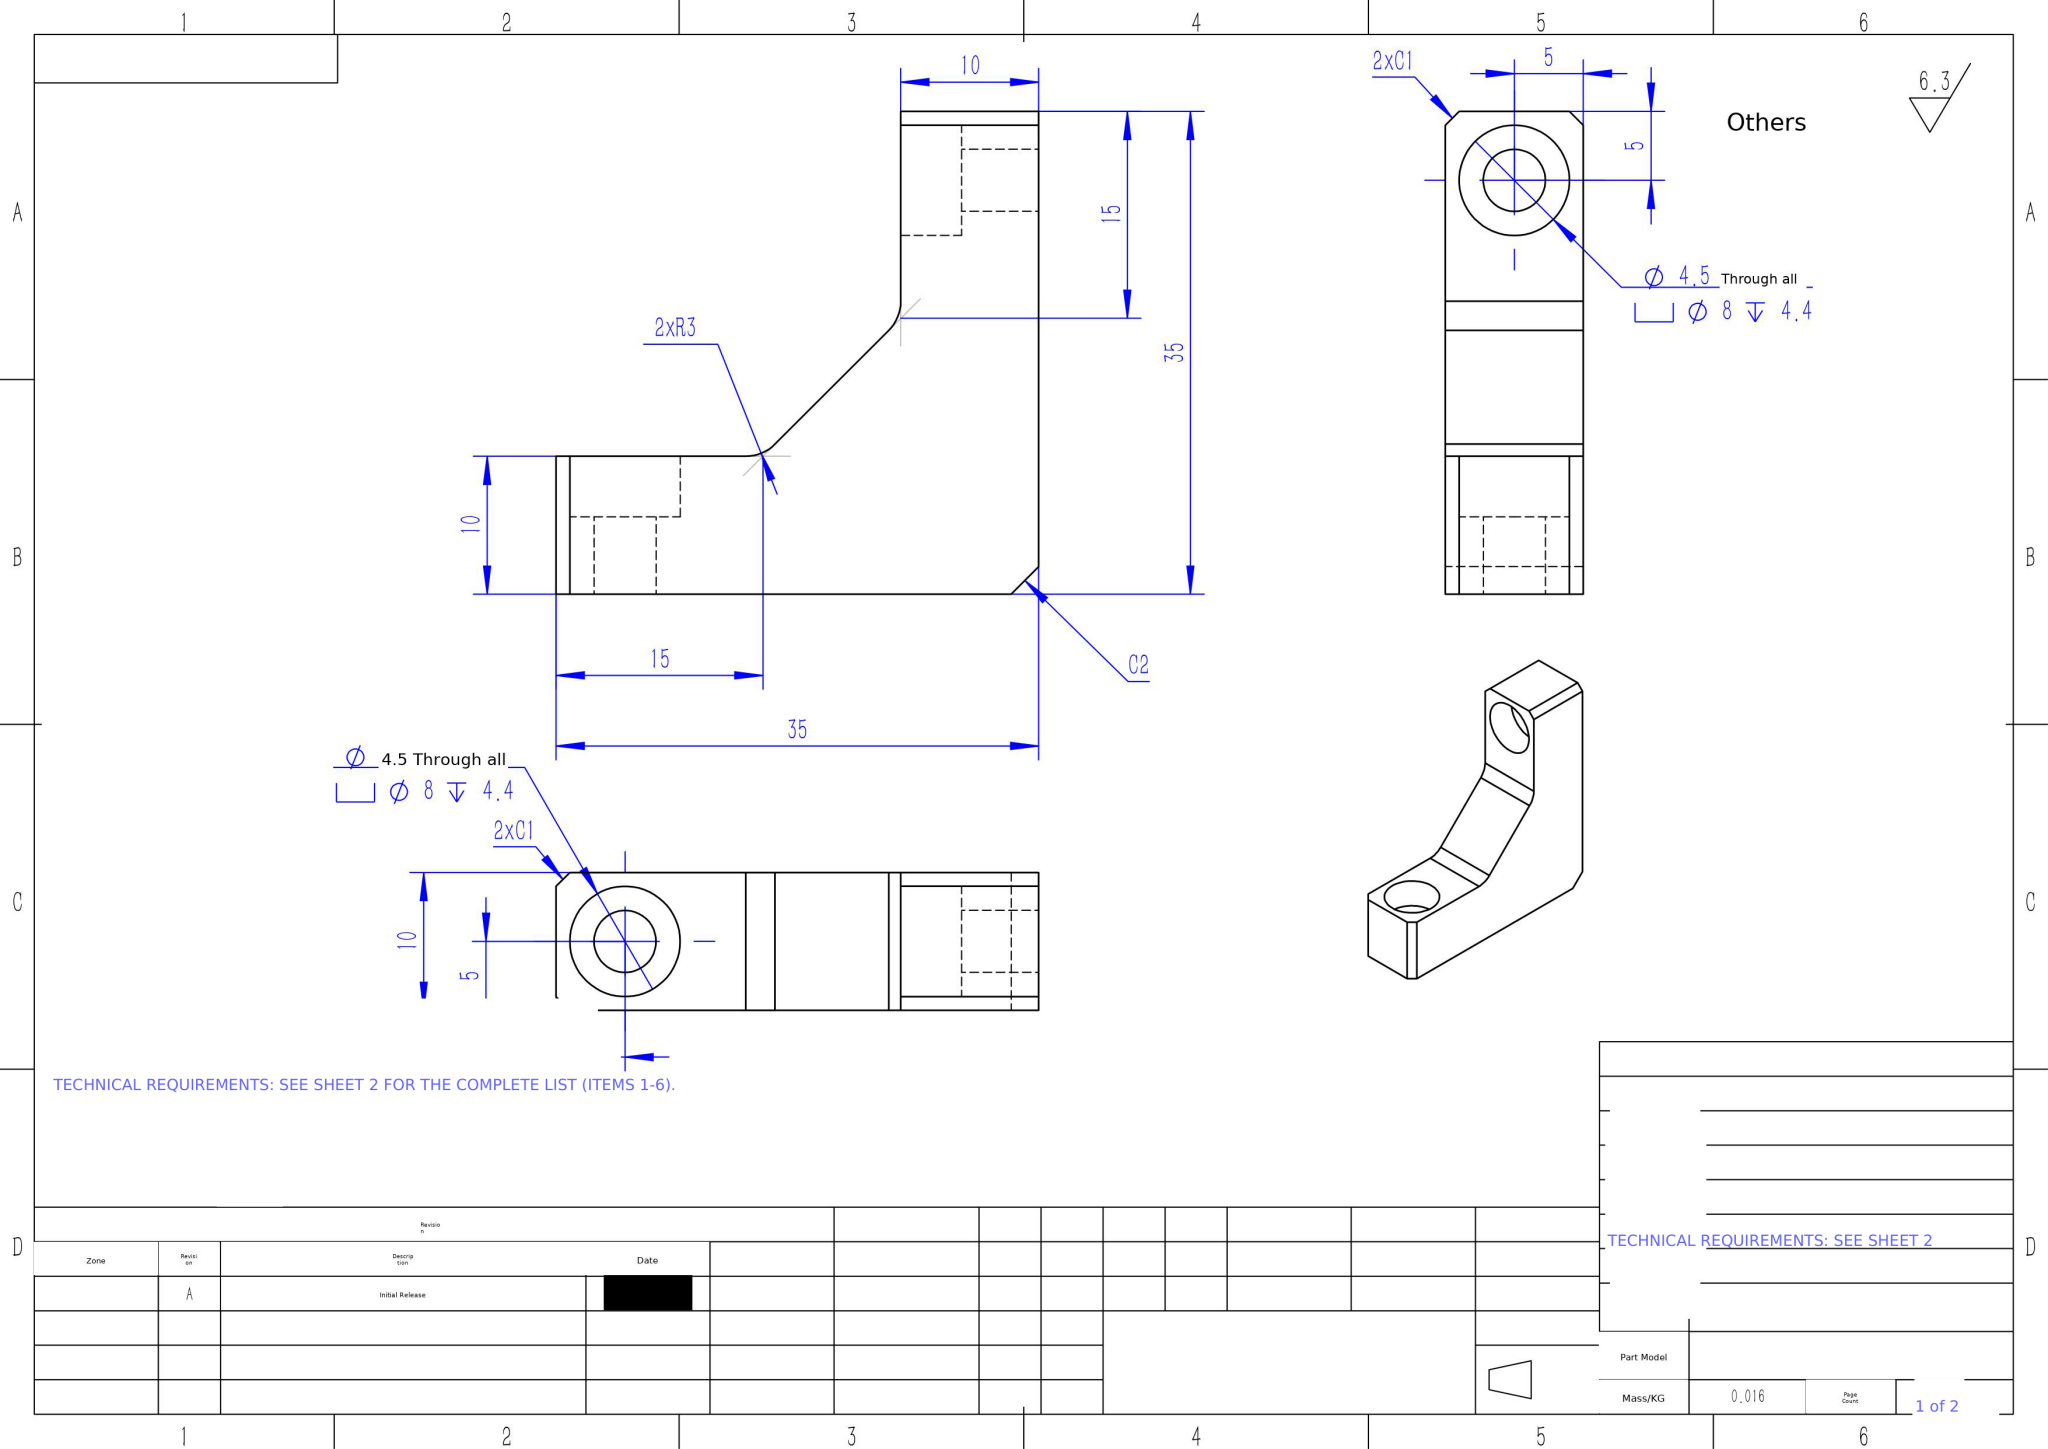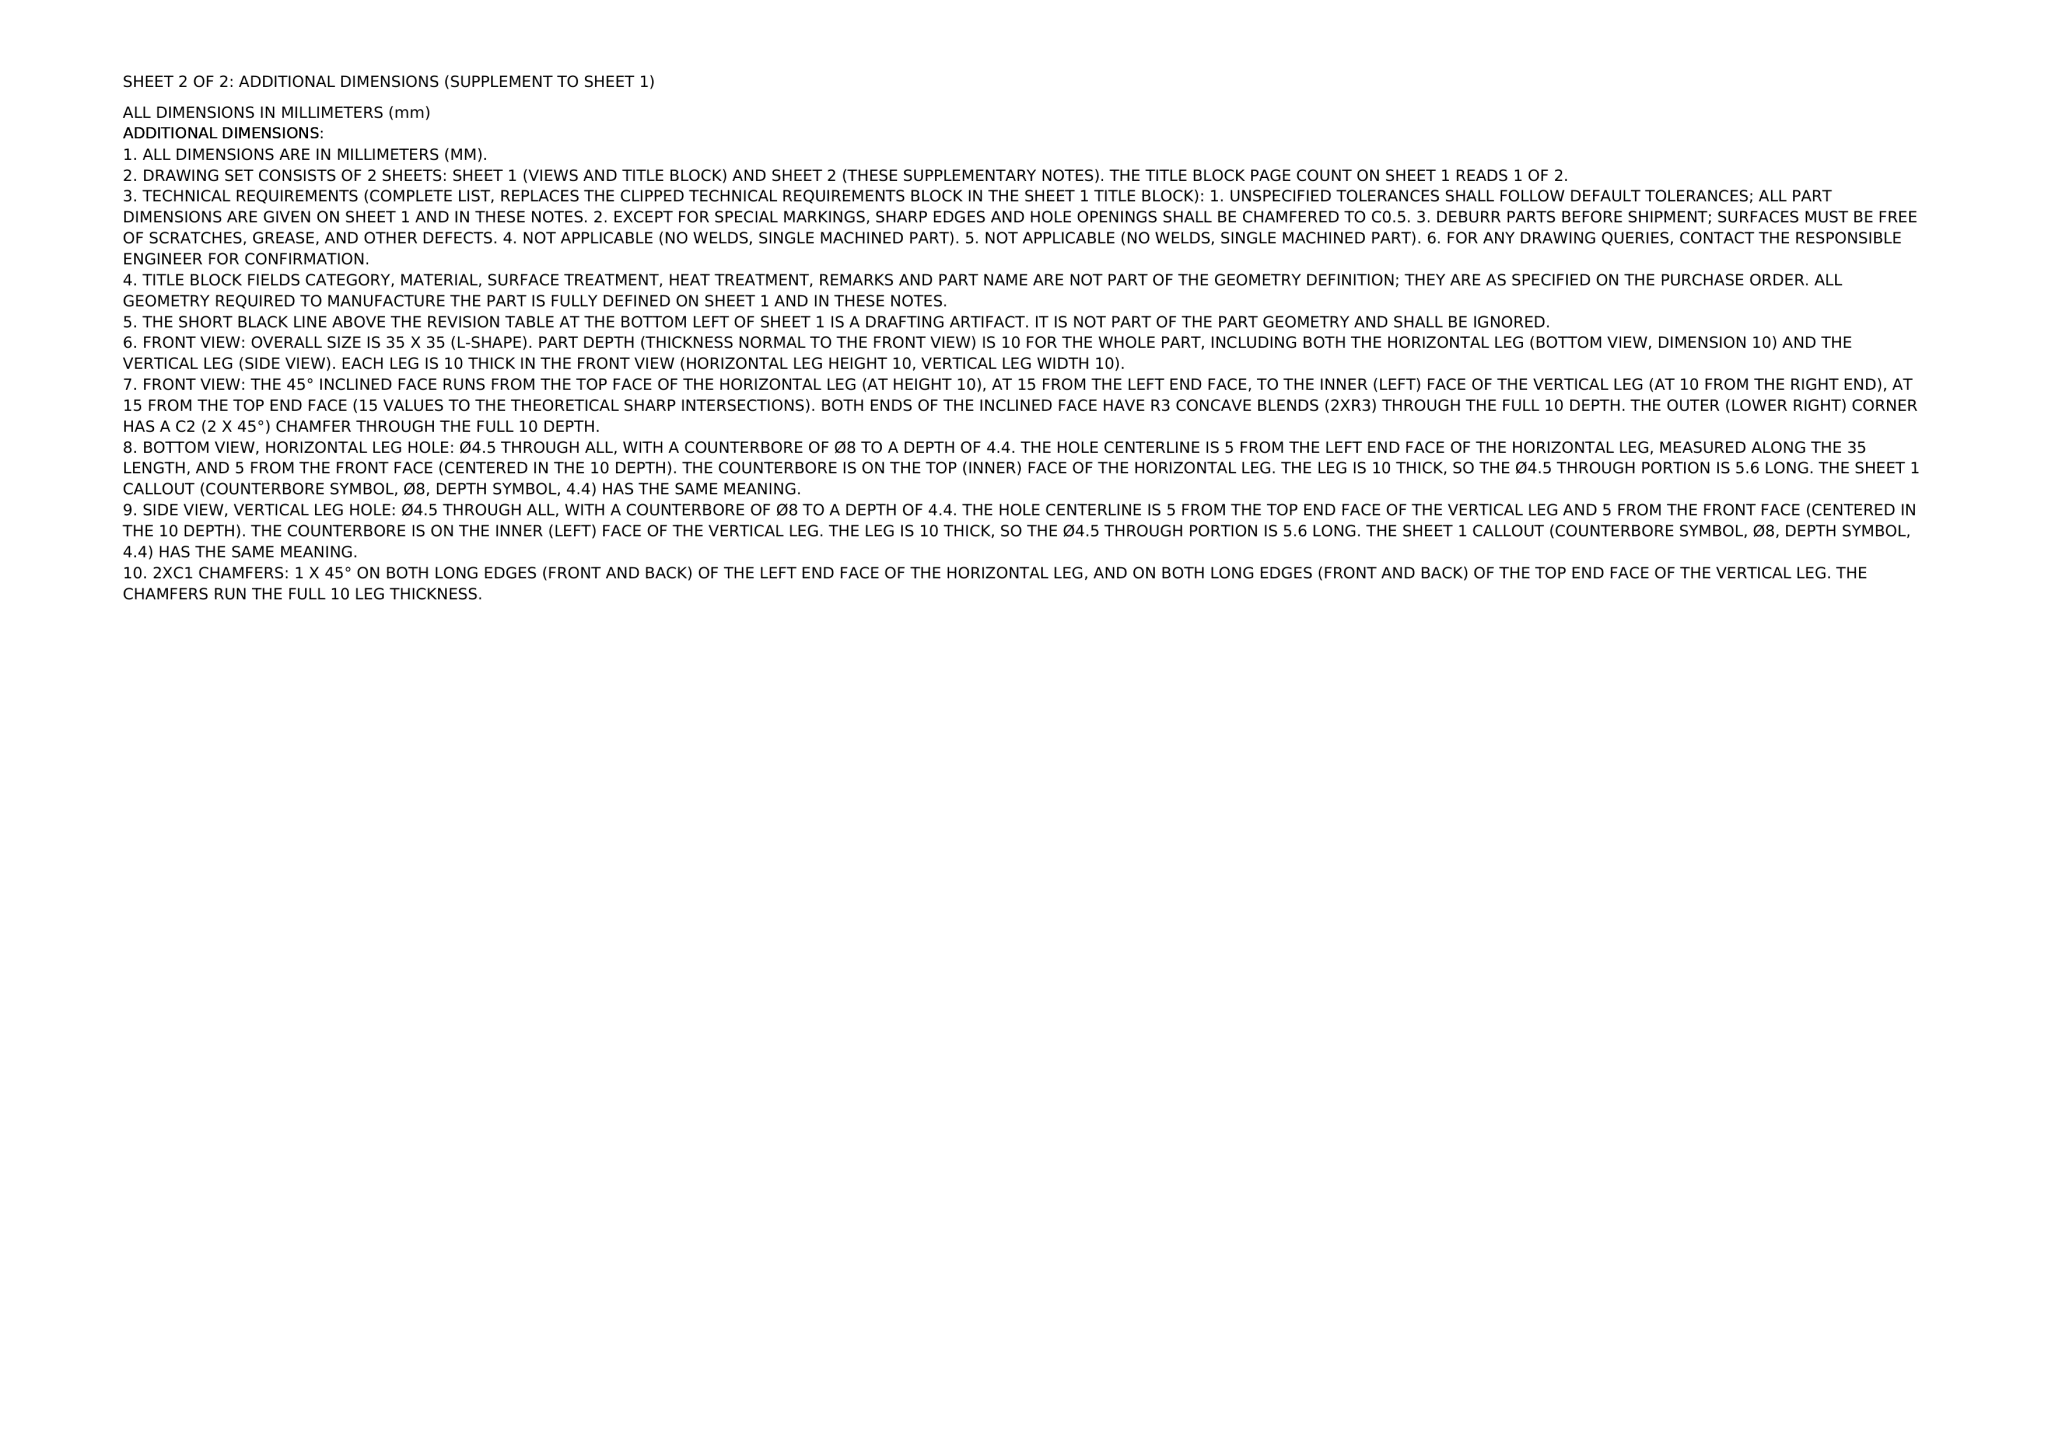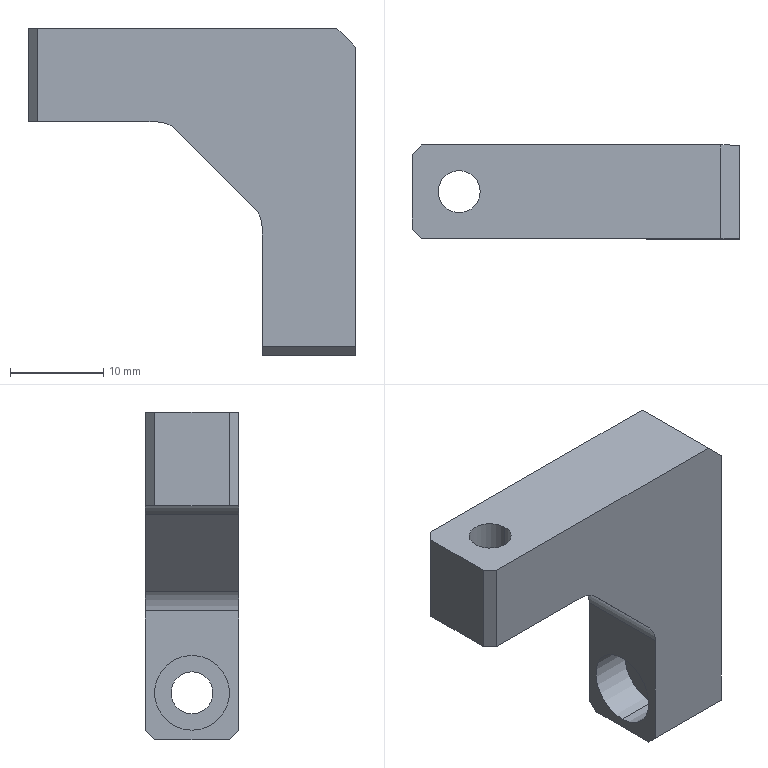Part | NX | mm | 1 solid | 26 faces | box 35 x 10 x 35 mm | volume 5843 mm3 | plane 16 | cylinder 10 | commonest cylinder face diameters 8 x4 4.5 x4 6 x2
STEP:
#1=COLOUR_RGB('',0.251,0.251,0.251);
#2=FILL_AREA_STYLE_COLOUR('',#1);
#3=FILL_AREA_STYLE('',(#2));
#4=SURFACE_STYLE_FILL_AREA(#3);
#5=SURFACE_SIDE_STYLE('',(#4));
#6=SURFACE_STYLE_USAGE(.BOTH.,#5);
#7=PRESENTATION_STYLE_ASSIGNMENT((#6));
#8=CARTESIAN_POINT('',(11.9,5.,-16.5));
#9=VERTEX_POINT('',#8);
#10=CARTESIAN_POINT('',(11.9,5.,-8.5));
#11=VERTEX_POINT('',#10);
#12=CARTESIAN_POINT('',(11.9,5.,-12.5));
#13=DIRECTION('',(-1.,0.,0.));
#14=DIRECTION('',(0.,0.,1.));
#15=AXIS2_PLACEMENT_3D('',#12,#13,#14);
#16=CIRCLE('',#15,4.);
#17=EDGE_CURVE('',#9,#11,#16,.T.);
#18=ORIENTED_EDGE('',*,*,#17,.F.);
#19=CARTESIAN_POINT('',(7.5,5.,-16.5));
#20=VERTEX_POINT('',#19);
#21=CARTESIAN_POINT('',(7.5,5.,-16.5));
#22=DIRECTION('',(-1.,0.,0.));
#23=VECTOR('',#22,1000.);
#24=LINE('',#21,#23);
#25=EDGE_CURVE('',#9,#20,#24,.T.);
#26=ORIENTED_EDGE('',*,*,#25,.T.);
#27=CARTESIAN_POINT('',(7.5,5.,-8.5));
#28=VERTEX_POINT('',#27);
#29=CARTESIAN_POINT('',(7.5,5.,-12.5));
#30=DIRECTION('',(-1.,0.,0.));
#31=DIRECTION('',(0.,0.,1.));
#32=AXIS2_PLACEMENT_3D('',#29,#30,#31);
#33=CIRCLE('',#32,4.);
#34=EDGE_CURVE('',#20,#28,#33,.T.);
#35=ORIENTED_EDGE('',*,*,#34,.T.);
#36=CARTESIAN_POINT('',(7.5,5.,-8.5));
#37=DIRECTION('',(-1.,0.,0.));
#38=VECTOR('',#37,1000.);
#39=LINE('',#36,#38);
#40=EDGE_CURVE('',#11,#28,#39,.T.);
#41=ORIENTED_EDGE('',*,*,#40,.F.);
#42=EDGE_LOOP('',(#18,#26,#35,#41));
#43=FACE_OUTER_BOUND('',#42,.T.);
#44=CARTESIAN_POINT('',(7.5,5.,-12.5));
#45=DIRECTION('',(-1.,0.,0.));
#46=DIRECTION('',(0.,0.,1.));
#47=AXIS2_PLACEMENT_3D('',#44,#45,#46);
#48=CYLINDRICAL_SURFACE('',#47,4.);
#49=ADVANCED_FACE('',(#43),#48,.F.);
#50=CARTESIAN_POINT('',(17.5,5.,-14.75));
#51=VERTEX_POINT('',#50);
#52=CARTESIAN_POINT('',(17.5,5.,-10.25));
#53=VERTEX_POINT('',#52);
#54=CARTESIAN_POINT('',(17.5,5.,-12.5));
#55=DIRECTION('',(-1.,0.,0.));
#56=DIRECTION('',(0.,0.,1.));
#57=AXIS2_PLACEMENT_3D('',#54,#55,#56);
#58=CIRCLE('',#57,2.25);
#59=EDGE_CURVE('',#51,#53,#58,.T.);
#60=ORIENTED_EDGE('',*,*,#59,.F.);
#61=CARTESIAN_POINT('',(11.9,5.,-14.75));
#62=VERTEX_POINT('',#61);
#63=CARTESIAN_POINT('',(7.5,5.,-14.75));
#64=DIRECTION('',(-1.,0.,0.));
#65=VECTOR('',#64,1000.);
#66=LINE('',#63,#65);
#67=EDGE_CURVE('',#51,#62,#66,.T.);
#68=ORIENTED_EDGE('',*,*,#67,.T.);
#69=CARTESIAN_POINT('',(11.9,5.,-10.25));
#70=VERTEX_POINT('',#69);
#71=CARTESIAN_POINT('',(11.9,5.,-12.5));
#72=DIRECTION('',(-1.,0.,0.));
#73=DIRECTION('',(0.,0.,1.));
#74=AXIS2_PLACEMENT_3D('',#71,#72,#73);
#75=CIRCLE('',#74,2.25);
#76=EDGE_CURVE('',#62,#70,#75,.T.);
#77=ORIENTED_EDGE('',*,*,#76,.T.);
#78=CARTESIAN_POINT('',(7.5,5.,-10.25));
#79=DIRECTION('',(-1.,0.,0.));
#80=VECTOR('',#79,1000.);
#81=LINE('',#78,#80);
#82=EDGE_CURVE('',#53,#70,#81,.T.);
#83=ORIENTED_EDGE('',*,*,#82,.F.);
#84=EDGE_LOOP('',(#60,#68,#77,#83));
#85=FACE_OUTER_BOUND('',#84,.T.);
#86=CARTESIAN_POINT('',(7.5,5.,-12.5));
#87=DIRECTION('',(-1.,0.,0.));
#88=DIRECTION('',(0.,0.,1.));
#89=AXIS2_PLACEMENT_3D('',#86,#87,#88);
#90=CYLINDRICAL_SURFACE('',#89,2.25);
#91=ADVANCED_FACE('',(#85),#90,.F.);
#92=CARTESIAN_POINT('',(-8.5,5.,11.9));
#93=VERTEX_POINT('',#92);
#94=CARTESIAN_POINT('',(-16.5,5.,11.9));
#95=VERTEX_POINT('',#94);
#96=CARTESIAN_POINT('',(-12.5,5.,11.9));
#97=DIRECTION('',(0.,0.,-1.));
#98=DIRECTION('',(-1.,0.,0.));
#99=AXIS2_PLACEMENT_3D('',#96,#97,#98);
#100=CIRCLE('',#99,4.);
#101=EDGE_CURVE('',#93,#95,#100,.T.);
#102=ORIENTED_EDGE('',*,*,#101,.F.);
#103=CARTESIAN_POINT('',(-8.5,5.,7.5));
#104=VERTEX_POINT('',#103);
#105=CARTESIAN_POINT('',(-8.5,5.,7.5));
#106=DIRECTION('',(0.,0.,-1.));
#107=VECTOR('',#106,1000.);
#108=LINE('',#105,#107);
#109=EDGE_CURVE('',#93,#104,#108,.T.);
#110=ORIENTED_EDGE('',*,*,#109,.T.);
#111=CARTESIAN_POINT('',(-16.5,5.,7.5));
#112=VERTEX_POINT('',#111);
#113=CARTESIAN_POINT('',(-12.5,5.,7.5));
#114=DIRECTION('',(0.,0.,-1.));
#115=DIRECTION('',(-1.,0.,0.));
#116=AXIS2_PLACEMENT_3D('',#113,#114,#115);
#117=CIRCLE('',#116,4.);
#118=EDGE_CURVE('',#104,#112,#117,.T.);
#119=ORIENTED_EDGE('',*,*,#118,.T.);
#120=CARTESIAN_POINT('',(-16.5,5.,7.5));
#121=DIRECTION('',(0.,0.,-1.));
#122=VECTOR('',#121,1000.);
#123=LINE('',#120,#122);
#124=EDGE_CURVE('',#95,#112,#123,.T.);
#125=ORIENTED_EDGE('',*,*,#124,.F.);
#126=EDGE_LOOP('',(#102,#110,#119,#125));
#127=FACE_OUTER_BOUND('',#126,.T.);
#128=CARTESIAN_POINT('',(-12.5,5.,7.5));
#129=DIRECTION('',(0.,0.,-1.));
#130=DIRECTION('',(-1.,0.,0.));
#131=AXIS2_PLACEMENT_3D('',#128,#129,#130);
#132=CYLINDRICAL_SURFACE('',#131,4.);
#133=ADVANCED_FACE('',(#127),#132,.F.);
#134=CARTESIAN_POINT('',(-10.25,5.,17.5));
#135=VERTEX_POINT('',#134);
#136=CARTESIAN_POINT('',(-14.75,5.,17.5));
#137=VERTEX_POINT('',#136);
#138=CARTESIAN_POINT('',(-12.5,5.,17.5));
#139=DIRECTION('',(0.,0.,-1.));
#140=DIRECTION('',(-1.,0.,0.));
#141=AXIS2_PLACEMENT_3D('',#138,#139,#140);
#142=CIRCLE('',#141,2.25);
#143=EDGE_CURVE('',#135,#137,#142,.T.);
#144=ORIENTED_EDGE('',*,*,#143,.F.);
#145=CARTESIAN_POINT('',(-10.25,5.,11.9));
#146=VERTEX_POINT('',#145);
#147=CARTESIAN_POINT('',(-10.25,5.,7.5));
#148=DIRECTION('',(0.,0.,-1.));
#149=VECTOR('',#148,1000.);
#150=LINE('',#147,#149);
#151=EDGE_CURVE('',#135,#146,#150,.T.);
#152=ORIENTED_EDGE('',*,*,#151,.T.);
#153=CARTESIAN_POINT('',(-14.75,5.,11.9));
#154=VERTEX_POINT('',#153);
#155=CARTESIAN_POINT('',(-12.5,5.,11.9));
#156=DIRECTION('',(0.,0.,-1.));
#157=DIRECTION('',(-1.,0.,0.));
#158=AXIS2_PLACEMENT_3D('',#155,#156,#157);
#159=CIRCLE('',#158,2.25);
#160=EDGE_CURVE('',#146,#154,#159,.T.);
#161=ORIENTED_EDGE('',*,*,#160,.T.);
#162=CARTESIAN_POINT('',(-14.75,5.,7.5));
#163=DIRECTION('',(0.,0.,-1.));
#164=VECTOR('',#163,1000.);
#165=LINE('',#162,#164);
#166=EDGE_CURVE('',#137,#154,#165,.T.);
#167=ORIENTED_EDGE('',*,*,#166,.F.);
#168=EDGE_LOOP('',(#144,#152,#161,#167));
#169=FACE_OUTER_BOUND('',#168,.T.);
#170=CARTESIAN_POINT('',(-12.5,5.,7.5));
#171=DIRECTION('',(0.,0.,-1.));
#172=DIRECTION('',(-1.,0.,0.));
#173=AXIS2_PLACEMENT_3D('',#170,#171,#172);
#174=CYLINDRICAL_SURFACE('',#173,2.25);
#175=ADVANCED_FACE('',(#169),#174,.F.);
#176=CARTESIAN_POINT('',(-17.5,1.,7.5));
#177=VERTEX_POINT('',#176);
#178=CARTESIAN_POINT('',(-17.5,9.,7.5));
#179=VERTEX_POINT('',#178);
#180=CARTESIAN_POINT('',(-17.5,0.,7.5));
#181=DIRECTION('',(0.,1.,0.));
#182=VECTOR('',#181,1000.);
#183=LINE('',#180,#182);
#184=EDGE_CURVE('',#177,#179,#183,.T.);
#185=ORIENTED_EDGE('',*,*,#184,.F.);
#186=CARTESIAN_POINT('',(-17.5,1.,17.5));
#187=VERTEX_POINT('',#186);
#188=CARTESIAN_POINT('',(-17.5,1.,17.5));
#189=DIRECTION('',(0.,0.,1.));
#190=VECTOR('',#189,1000.);
#191=LINE('',#188,#190);
#192=EDGE_CURVE('',#177,#187,#191,.T.);
#193=ORIENTED_EDGE('',*,*,#192,.T.);
#194=CARTESIAN_POINT('',(-17.5,9.,17.5));
#195=VERTEX_POINT('',#194);
#196=CARTESIAN_POINT('',(-17.5,10.,17.5));
#197=DIRECTION('',(0.,-1.,0.));
#198=VECTOR('',#197,1000.);
#199=LINE('',#196,#198);
#200=EDGE_CURVE('',#195,#187,#199,.T.);
#201=ORIENTED_EDGE('',*,*,#200,.F.);
#202=CARTESIAN_POINT('',(-17.5,9.,7.5));
#203=DIRECTION('',(0.,0.,-1.));
#204=VECTOR('',#203,1000.);
#205=LINE('',#202,#204);
#206=EDGE_CURVE('',#195,#179,#205,.T.);
#207=ORIENTED_EDGE('',*,*,#206,.T.);
#208=EDGE_LOOP('',(#185,#193,#201,#207));
#209=FACE_OUTER_BOUND('',#208,.T.);
#210=CARTESIAN_POINT('',(-17.5,10.,17.5));
#211=DIRECTION('',(1.,0.,0.));
#212=DIRECTION('',(0.,0.,-1.));
#213=AXIS2_PLACEMENT_3D('',#210,#211,#212);
#214=PLANE('',#213);
#215=ADVANCED_FACE('',(#209),#214,.F.);
#216=CARTESIAN_POINT('',(-12.5,5.,17.5));
#217=DIRECTION('',(0.,0.,-1.));
#218=DIRECTION('',(-1.,0.,0.));
#219=AXIS2_PLACEMENT_3D('',#216,#217,#218);
#220=CIRCLE('',#219,2.25);
#221=EDGE_CURVE('',#137,#135,#220,.T.);
#222=ORIENTED_EDGE('',*,*,#221,.T.);
#223=ORIENTED_EDGE('',*,*,#143,.T.);
#224=EDGE_LOOP('',(#222,#223));
#225=FACE_BOUND('',#224,.T.);
#226=ORIENTED_EDGE('',*,*,#200,.T.);
#227=CARTESIAN_POINT('',(-16.5,0.,17.5));
#228=VERTEX_POINT('',#227);
#229=CARTESIAN_POINT('',(-17.5,1.,17.5));
#230=DIRECTION('',(0.7071,-0.7071,-0.));
#231=VECTOR('',#230,1000.);
#232=LINE('',#229,#231);
#233=EDGE_CURVE('',#187,#228,#232,.T.);
#234=ORIENTED_EDGE('',*,*,#233,.T.);
#235=CARTESIAN_POINT('',(15.5,0.,17.5));
#236=VERTEX_POINT('',#235);
#237=CARTESIAN_POINT('',(17.5,0.,17.5));
#238=DIRECTION('',(1.,0.,-0.));
#239=VECTOR('',#238,1000.);
#240=LINE('',#237,#239);
#241=EDGE_CURVE('',#228,#236,#240,.T.);
#242=ORIENTED_EDGE('',*,*,#241,.T.);
#243=CARTESIAN_POINT('',(15.5,10.,17.5));
#244=VERTEX_POINT('',#243);
#245=CARTESIAN_POINT('',(15.5,10.,17.5));
#246=DIRECTION('',(0.,1.,0.));
#247=VECTOR('',#246,1000.);
#248=LINE('',#245,#247);
#249=EDGE_CURVE('',#236,#244,#248,.T.);
#250=ORIENTED_EDGE('',*,*,#249,.T.);
#251=CARTESIAN_POINT('',(-16.5,10.,17.5));
#252=VERTEX_POINT('',#251);
#253=CARTESIAN_POINT('',(17.5,10.,17.5));
#254=DIRECTION('',(1.,0.,-0.));
#255=VECTOR('',#254,1000.);
#256=LINE('',#253,#255);
#257=EDGE_CURVE('',#252,#244,#256,.T.);
#258=ORIENTED_EDGE('',*,*,#257,.F.);
#259=CARTESIAN_POINT('',(-16.5,10.,17.5));
#260=DIRECTION('',(-0.7071,-0.7071,0.));
#261=VECTOR('',#260,1000.);
#262=LINE('',#259,#261);
#263=EDGE_CURVE('',#252,#195,#262,.T.);
#264=ORIENTED_EDGE('',*,*,#263,.T.);
#265=EDGE_LOOP('',(#226,#234,#242,#250,#258,#264));
#266=FACE_OUTER_BOUND('',#265,.T.);
#267=CARTESIAN_POINT('',(17.5,10.,17.5));
#268=DIRECTION('',(-0.,0.,-1.));
#269=DIRECTION('',(-1.,0.,0.));
#270=AXIS2_PLACEMENT_3D('',#267,#268,#269);
#271=PLANE('',#270);
#272=ADVANCED_FACE('',(#225,#266),#271,.F.);
#273=CARTESIAN_POINT('',(17.5,5.,-12.5));
#274=DIRECTION('',(-1.,0.,0.));
#275=DIRECTION('',(0.,0.,1.));
#276=AXIS2_PLACEMENT_3D('',#273,#274,#275);
#277=CIRCLE('',#276,2.25);
#278=EDGE_CURVE('',#53,#51,#277,.T.);
#279=ORIENTED_EDGE('',*,*,#278,.T.);
#280=ORIENTED_EDGE('',*,*,#59,.T.);
#281=EDGE_LOOP('',(#279,#280));
#282=FACE_BOUND('',#281,.T.);
#283=CARTESIAN_POINT('',(17.5,9.,-17.5));
#284=VERTEX_POINT('',#283);
#285=CARTESIAN_POINT('',(17.5,1.,-17.5));
#286=VERTEX_POINT('',#285);
#287=CARTESIAN_POINT('',(17.5,10.,-17.5));
#288=DIRECTION('',(0.,-1.,0.));
#289=VECTOR('',#288,1000.);
#290=LINE('',#287,#289);
#291=EDGE_CURVE('',#284,#286,#290,.T.);
#292=ORIENTED_EDGE('',*,*,#291,.F.);
#293=CARTESIAN_POINT('',(17.5,10.,-16.5));
#294=VERTEX_POINT('',#293);
#295=CARTESIAN_POINT('',(17.5,10.,-16.5));
#296=DIRECTION('',(0.,0.7071,0.7071));
#297=VECTOR('',#296,1000.);
#298=LINE('',#295,#297);
#299=EDGE_CURVE('',#284,#294,#298,.T.);
#300=ORIENTED_EDGE('',*,*,#299,.T.);
#301=CARTESIAN_POINT('',(17.5,10.,15.5));
#302=VERTEX_POINT('',#301);
#303=CARTESIAN_POINT('',(17.5,10.,17.5));
#304=DIRECTION('',(0.,0.,-1.));
#305=VECTOR('',#304,1000.);
#306=LINE('',#303,#305);
#307=EDGE_CURVE('',#302,#294,#306,.T.);
#308=ORIENTED_EDGE('',*,*,#307,.F.);
#309=CARTESIAN_POINT('',(17.5,0.,15.5));
#310=VERTEX_POINT('',#309);
#311=CARTESIAN_POINT('',(17.5,10.,15.5));
#312=DIRECTION('',(0.,-1.,0.));
#313=VECTOR('',#312,1000.);
#314=LINE('',#311,#313);
#315=EDGE_CURVE('',#302,#310,#314,.T.);
#316=ORIENTED_EDGE('',*,*,#315,.T.);
#317=CARTESIAN_POINT('',(17.5,0.,-16.5));
#318=VERTEX_POINT('',#317);
#319=CARTESIAN_POINT('',(17.5,0.,17.5));
#320=DIRECTION('',(0.,0.,-1.));
#321=VECTOR('',#320,1000.);
#322=LINE('',#319,#321);
#323=EDGE_CURVE('',#310,#318,#322,.T.);
#324=ORIENTED_EDGE('',*,*,#323,.T.);
#325=CARTESIAN_POINT('',(17.5,1.,-17.5));
#326=DIRECTION('',(0.,0.7071,-0.7071));
#327=VECTOR('',#326,1000.);
#328=LINE('',#325,#327);
#329=EDGE_CURVE('',#318,#286,#328,.T.);
#330=ORIENTED_EDGE('',*,*,#329,.T.);
#331=EDGE_LOOP('',(#292,#300,#308,#316,#324,#330));
#332=FACE_OUTER_BOUND('',#331,.T.);
#333=CARTESIAN_POINT('',(17.5,10.,17.5));
#334=DIRECTION('',(-1.,0.,0.));
#335=DIRECTION('',(0.,0.,1.));
#336=AXIS2_PLACEMENT_3D('',#333,#334,#335);
#337=PLANE('',#336);
#338=ADVANCED_FACE('',(#282,#332),#337,.F.);
#339=CARTESIAN_POINT('',(7.5,1.,-17.5));
#340=VERTEX_POINT('',#339);
#341=CARTESIAN_POINT('',(7.5,9.,-17.5));
#342=VERTEX_POINT('',#341);
#343=CARTESIAN_POINT('',(7.5,0.,-17.5));
#344=DIRECTION('',(0.,1.,0.));
#345=VECTOR('',#344,1000.);
#346=LINE('',#343,#345);
#347=EDGE_CURVE('',#340,#342,#346,.T.);
#348=ORIENTED_EDGE('',*,*,#347,.T.);
#349=CARTESIAN_POINT('',(17.5,9.,-17.5));
#350=DIRECTION('',(1.,0.,-0.));
#351=VECTOR('',#350,1000.);
#352=LINE('',#349,#351);
#353=EDGE_CURVE('',#342,#284,#352,.T.);
#354=ORIENTED_EDGE('',*,*,#353,.T.);
#355=ORIENTED_EDGE('',*,*,#291,.T.);
#356=CARTESIAN_POINT('',(17.5,1.,-17.5));
#357=DIRECTION('',(-1.,0.,0.));
#358=VECTOR('',#357,1000.);
#359=LINE('',#356,#358);
#360=EDGE_CURVE('',#286,#340,#359,.T.);
#361=ORIENTED_EDGE('',*,*,#360,.T.);
#362=EDGE_LOOP('',(#348,#354,#355,#361));
#363=FACE_OUTER_BOUND('',#362,.T.);
#364=CARTESIAN_POINT('',(17.5,10.,-17.5));
#365=DIRECTION('',(0.,0.,1.));
#366=DIRECTION('',(1.,0.,-0.));
#367=AXIS2_PLACEMENT_3D('',#364,#365,#366);
#368=PLANE('',#367);
#369=ADVANCED_FACE('',(#363),#368,.F.);
#370=ORIENTED_EDGE('',*,*,#307,.T.);
#371=CARTESIAN_POINT('',(7.5,10.,-16.5));
#372=VERTEX_POINT('',#371);
#373=CARTESIAN_POINT('',(7.5,10.,-16.5));
#374=DIRECTION('',(-1.,0.,0.));
#375=VECTOR('',#374,1000.);
#376=LINE('',#373,#375);
#377=EDGE_CURVE('',#294,#372,#376,.T.);
#378=ORIENTED_EDGE('',*,*,#377,.T.);
#379=CARTESIAN_POINT('',(7.5,10.,-3.743));
#380=VERTEX_POINT('',#379);
#381=CARTESIAN_POINT('',(7.5,10.,-2.5));
#382=DIRECTION('',(0.,0.,-1.));
#383=VECTOR('',#382,1000.);
#384=LINE('',#381,#383);
#385=EDGE_CURVE('',#380,#372,#384,.T.);
#386=ORIENTED_EDGE('',*,*,#385,.F.);
#387=CARTESIAN_POINT('',(6.621,10.,-1.621));
#388=VERTEX_POINT('',#387);
#389=CARTESIAN_POINT('',(4.5,10.,-3.743));
#390=DIRECTION('',(0.,-1.,0.));
#391=DIRECTION('',(-0.,0.,1.));
#392=AXIS2_PLACEMENT_3D('',#389,#390,#391);
#393=CIRCLE('',#392,3.);
#394=EDGE_CURVE('',#380,#388,#393,.T.);
#395=ORIENTED_EDGE('',*,*,#394,.T.);
#396=CARTESIAN_POINT('',(-1.621,10.,6.621));
#397=VERTEX_POINT('',#396);
#398=CARTESIAN_POINT('',(7.5,10.,-2.5));
#399=DIRECTION('',(0.7071,0.,-0.7071));
#400=VECTOR('',#399,1000.);
#401=LINE('',#398,#400);
#402=EDGE_CURVE('',#397,#388,#401,.T.);
#403=ORIENTED_EDGE('',*,*,#402,.F.);
#404=CARTESIAN_POINT('',(-3.743,10.,7.5));
#405=VERTEX_POINT('',#404);
#406=CARTESIAN_POINT('',(-3.743,10.,4.5));
#407=DIRECTION('',(0.,-1.,0.));
#408=DIRECTION('',(0.,0.,1.));
#409=AXIS2_PLACEMENT_3D('',#406,#407,#408);
#410=CIRCLE('',#409,3.);
#411=EDGE_CURVE('',#397,#405,#410,.T.);
#412=ORIENTED_EDGE('',*,*,#411,.T.);
#413=CARTESIAN_POINT('',(-16.5,10.,7.5));
#414=VERTEX_POINT('',#413);
#415=CARTESIAN_POINT('',(-17.5,10.,7.5));
#416=DIRECTION('',(1.,0.,0.));
#417=VECTOR('',#416,1000.);
#418=LINE('',#415,#417);
#419=EDGE_CURVE('',#414,#405,#418,.T.);
#420=ORIENTED_EDGE('',*,*,#419,.F.);
#421=CARTESIAN_POINT('',(-16.5,10.,17.5));
#422=DIRECTION('',(0.,0.,1.));
#423=VECTOR('',#422,1000.);
#424=LINE('',#421,#423);
#425=EDGE_CURVE('',#414,#252,#424,.T.);
#426=ORIENTED_EDGE('',*,*,#425,.T.);
#427=ORIENTED_EDGE('',*,*,#257,.T.);
#428=CARTESIAN_POINT('',(16.5,10.,16.5));
#429=DIRECTION('',(0.7071,0.,-0.7071));
#430=VECTOR('',#429,1000.);
#431=LINE('',#428,#430);
#432=EDGE_CURVE('',#244,#302,#431,.T.);
#433=ORIENTED_EDGE('',*,*,#432,.T.);
#434=EDGE_LOOP('',(#370,#378,#386,#395,#403,#412,#420,#426,#427,#433));
#435=FACE_OUTER_BOUND('',#434,.T.);
#436=CARTESIAN_POINT('',(0.,10.,0.));
#437=DIRECTION('',(0.,1.,0.));
#438=DIRECTION('',(0.,0.,1.));
#439=AXIS2_PLACEMENT_3D('',#436,#437,#438);
#440=PLANE('',#439);
#441=ADVANCED_FACE('',(#435),#440,.T.);
#442=CARTESIAN_POINT('',(-1.621,0.,6.621));
#443=VERTEX_POINT('',#442);
#444=CARTESIAN_POINT('',(6.621,0.,-1.621));
#445=VERTEX_POINT('',#444);
#446=CARTESIAN_POINT('',(7.5,0.,-2.5));
#447=DIRECTION('',(0.7071,0.,-0.7071));
#448=VECTOR('',#447,1000.);
#449=LINE('',#446,#448);
#450=EDGE_CURVE('',#443,#445,#449,.T.);
#451=ORIENTED_EDGE('',*,*,#450,.T.);
#452=CARTESIAN_POINT('',(7.5,0.,-3.743));
#453=VERTEX_POINT('',#452);
#454=CARTESIAN_POINT('',(4.5,0.,-3.743));
#455=DIRECTION('',(0.,1.,0.));
#456=DIRECTION('',(0.,0.,1.));
#457=AXIS2_PLACEMENT_3D('',#454,#455,#456);
#458=CIRCLE('',#457,3.);
#459=EDGE_CURVE('',#445,#453,#458,.T.);
#460=ORIENTED_EDGE('',*,*,#459,.T.);
#461=CARTESIAN_POINT('',(7.5,0.,-16.5));
#462=VERTEX_POINT('',#461);
#463=CARTESIAN_POINT('',(7.5,0.,-2.5));
#464=DIRECTION('',(0.,0.,-1.));
#465=VECTOR('',#464,1000.);
#466=LINE('',#463,#465);
#467=EDGE_CURVE('',#453,#462,#466,.T.);
#468=ORIENTED_EDGE('',*,*,#467,.T.);
#469=CARTESIAN_POINT('',(-0.,0.,-16.5));
#470=DIRECTION('',(1.,0.,-0.));
#471=VECTOR('',#470,1000.);
#472=LINE('',#469,#471);
#473=EDGE_CURVE('',#462,#318,#472,.T.);
#474=ORIENTED_EDGE('',*,*,#473,.T.);
#475=ORIENTED_EDGE('',*,*,#323,.F.);
#476=CARTESIAN_POINT('',(17.5,0.,15.5));
#477=DIRECTION('',(-0.7071,0.,0.7071));
#478=VECTOR('',#477,1000.);
#479=LINE('',#476,#478);
#480=EDGE_CURVE('',#310,#236,#479,.T.);
#481=ORIENTED_EDGE('',*,*,#480,.T.);
#482=ORIENTED_EDGE('',*,*,#241,.F.);
#483=CARTESIAN_POINT('',(-16.5,0.,7.5));
#484=VERTEX_POINT('',#483);
#485=CARTESIAN_POINT('',(-16.5,0.,0.));
#486=DIRECTION('',(0.,0.,-1.));
#487=VECTOR('',#486,1000.);
#488=LINE('',#485,#487);
#489=EDGE_CURVE('',#228,#484,#488,.T.);
#490=ORIENTED_EDGE('',*,*,#489,.T.);
#491=CARTESIAN_POINT('',(-3.743,0.,7.5));
#492=VERTEX_POINT('',#491);
#493=CARTESIAN_POINT('',(-17.5,0.,7.5));
#494=DIRECTION('',(1.,0.,0.));
#495=VECTOR('',#494,1000.);
#496=LINE('',#493,#495);
#497=EDGE_CURVE('',#484,#492,#496,.T.);
#498=ORIENTED_EDGE('',*,*,#497,.T.);
#499=CARTESIAN_POINT('',(-3.743,0.,4.5));
#500=DIRECTION('',(0.,1.,0.));
#501=DIRECTION('',(0.,0.,1.));
#502=AXIS2_PLACEMENT_3D('',#499,#500,#501);
#503=CIRCLE('',#502,3.);
#504=EDGE_CURVE('',#492,#443,#503,.T.);
#505=ORIENTED_EDGE('',*,*,#504,.T.);
#506=EDGE_LOOP('',(#451,#460,#468,#474,#475,#481,#482,#490,#498,#505));
#507=FACE_OUTER_BOUND('',#506,.T.);
#508=CARTESIAN_POINT('',(0.,0.,0.));
#509=DIRECTION('',(0.,1.,0.));
#510=DIRECTION('',(0.,0.,1.));
#511=AXIS2_PLACEMENT_3D('',#508,#509,#510);
#512=PLANE('',#511);
#513=ADVANCED_FACE('',(#507),#512,.F.);
#514=CARTESIAN_POINT('',(7.5,5.,-12.5));
#515=DIRECTION('',(-1.,0.,0.));
#516=DIRECTION('',(0.,0.,1.));
#517=AXIS2_PLACEMENT_3D('',#514,#515,#516);
#518=CIRCLE('',#517,4.);
#519=EDGE_CURVE('',#28,#20,#518,.T.);
#520=ORIENTED_EDGE('',*,*,#519,.F.);
#521=ORIENTED_EDGE('',*,*,#34,.F.);
#522=EDGE_LOOP('',(#520,#521));
#523=FACE_BOUND('',#522,.T.);
#524=ORIENTED_EDGE('',*,*,#467,.F.);
#525=CARTESIAN_POINT('',(7.5,10.,-3.743));
#526=DIRECTION('',(0.,1.,0.));
#527=VECTOR('',#526,1000.);
#528=LINE('',#525,#527);
#529=EDGE_CURVE('',#453,#380,#528,.T.);
#530=ORIENTED_EDGE('',*,*,#529,.T.);
#531=ORIENTED_EDGE('',*,*,#385,.T.);
#532=CARTESIAN_POINT('',(7.5,10.,-16.5));
#533=DIRECTION('',(0.,-0.7071,-0.7071));
#534=VECTOR('',#533,1000.);
#535=LINE('',#532,#534);
#536=EDGE_CURVE('',#372,#342,#535,.T.);
#537=ORIENTED_EDGE('',*,*,#536,.T.);
#538=ORIENTED_EDGE('',*,*,#347,.F.);
#539=CARTESIAN_POINT('',(7.5,1.,-17.5));
#540=DIRECTION('',(0.,-0.7071,0.7071));
#541=VECTOR('',#540,1000.);
#542=LINE('',#539,#541);
#543=EDGE_CURVE('',#340,#462,#542,.T.);
#544=ORIENTED_EDGE('',*,*,#543,.T.);
#545=EDGE_LOOP('',(#524,#530,#531,#537,#538,#544));
#546=FACE_OUTER_BOUND('',#545,.T.);
#547=CARTESIAN_POINT('',(7.5,0.,-2.5));
#548=DIRECTION('',(1.,0.,0.));
#549=DIRECTION('',(0.,0.,-1.));
#550=AXIS2_PLACEMENT_3D('',#547,#548,#549);
#551=PLANE('',#550);
#552=ADVANCED_FACE('',(#523,#546),#551,.F.);
#553=ORIENTED_EDGE('',*,*,#402,.T.);
#554=CARTESIAN_POINT('',(6.621,0.,-1.621));
#555=DIRECTION('',(0.,-1.,0.));
#556=VECTOR('',#555,1000.);
#557=LINE('',#554,#556);
#558=EDGE_CURVE('',#388,#445,#557,.T.);
#559=ORIENTED_EDGE('',*,*,#558,.T.);
#560=ORIENTED_EDGE('',*,*,#450,.F.);
#561=CARTESIAN_POINT('',(-1.621,10.,6.621));
#562=DIRECTION('',(0.,1.,0.));
#563=VECTOR('',#562,1000.);
#564=LINE('',#561,#563);
#565=EDGE_CURVE('',#443,#397,#564,.T.);
#566=ORIENTED_EDGE('',*,*,#565,.T.);
#567=EDGE_LOOP('',(#553,#559,#560,#566));
#568=FACE_OUTER_BOUND('',#567,.T.);
#569=CARTESIAN_POINT('',(7.5,0.,-2.5));
#570=DIRECTION('',(0.7071,0.,0.7071));
#571=DIRECTION('',(0.7071,0.,-0.7071));
#572=AXIS2_PLACEMENT_3D('',#569,#570,#571);
#573=PLANE('',#572);
#574=ADVANCED_FACE('',(#568),#573,.F.);
#575=CARTESIAN_POINT('',(-12.5,5.,7.5));
#576=DIRECTION('',(0.,0.,-1.));
#577=DIRECTION('',(-1.,0.,0.));
#578=AXIS2_PLACEMENT_3D('',#575,#576,#577);
#579=CIRCLE('',#578,4.);
#580=EDGE_CURVE('',#112,#104,#579,.T.);
#581=ORIENTED_EDGE('',*,*,#580,.F.);
#582=ORIENTED_EDGE('',*,*,#118,.F.);
#583=EDGE_LOOP('',(#581,#582));
#584=FACE_BOUND('',#583,.T.);
#585=ORIENTED_EDGE('',*,*,#419,.T.);
#586=CARTESIAN_POINT('',(-3.743,0.,7.5));
#587=DIRECTION('',(0.,-1.,0.));
#588=VECTOR('',#587,1000.);
#589=LINE('',#586,#588);
#590=EDGE_CURVE('',#405,#492,#589,.T.);
#591=ORIENTED_EDGE('',*,*,#590,.T.);
#592=ORIENTED_EDGE('',*,*,#497,.F.);
#593=CARTESIAN_POINT('',(-17.5,1.,7.5));
#594=DIRECTION('',(-0.7071,0.7071,-0.));
#595=VECTOR('',#594,1000.);
#596=LINE('',#593,#595);
#597=EDGE_CURVE('',#484,#177,#596,.T.);
#598=ORIENTED_EDGE('',*,*,#597,.T.);
#599=ORIENTED_EDGE('',*,*,#184,.T.);
#600=CARTESIAN_POINT('',(-16.5,10.,7.5));
#601=DIRECTION('',(0.7071,0.7071,0.));
#602=VECTOR('',#601,1000.);
#603=LINE('',#600,#602);
#604=EDGE_CURVE('',#179,#414,#603,.T.);
#605=ORIENTED_EDGE('',*,*,#604,.T.);
#606=EDGE_LOOP('',(#585,#591,#592,#598,#599,#605));
#607=FACE_OUTER_BOUND('',#606,.T.);
#608=CARTESIAN_POINT('',(-17.5,0.,7.5));
#609=DIRECTION('',(-0.,0.,1.));
#610=DIRECTION('',(1.,0.,0.));
#611=AXIS2_PLACEMENT_3D('',#608,#609,#610);
#612=PLANE('',#611);
#613=ADVANCED_FACE('',(#584,#607),#612,.F.);
#614=ORIENTED_EDGE('',*,*,#151,.F.);
#615=ORIENTED_EDGE('',*,*,#221,.F.);
#616=ORIENTED_EDGE('',*,*,#166,.T.);
#617=CARTESIAN_POINT('',(-12.5,5.,11.9));
#618=DIRECTION('',(0.,0.,-1.));
#619=DIRECTION('',(-1.,0.,0.));
#620=AXIS2_PLACEMENT_3D('',#617,#618,#619);
#621=CIRCLE('',#620,2.25);
#622=EDGE_CURVE('',#154,#146,#621,.T.);
#623=ORIENTED_EDGE('',*,*,#622,.T.);
#624=EDGE_LOOP('',(#614,#615,#616,#623));
#625=FACE_OUTER_BOUND('',#624,.T.);
#626=CARTESIAN_POINT('',(-12.5,5.,7.5));
#627=DIRECTION('',(0.,0.,-1.));
#628=DIRECTION('',(-1.,0.,0.));
#629=AXIS2_PLACEMENT_3D('',#626,#627,#628);
#630=CYLINDRICAL_SURFACE('',#629,2.25);
#631=ADVANCED_FACE('',(#625),#630,.F.);
#632=ORIENTED_EDGE('',*,*,#622,.F.);
#633=ORIENTED_EDGE('',*,*,#160,.F.);
#634=EDGE_LOOP('',(#632,#633));
#635=FACE_BOUND('',#634,.T.);
#636=CARTESIAN_POINT('',(-12.5,5.,11.9));
#637=DIRECTION('',(0.,0.,-1.));
#638=DIRECTION('',(-1.,0.,0.));
#639=AXIS2_PLACEMENT_3D('',#636,#637,#638);
#640=CIRCLE('',#639,4.);
#641=EDGE_CURVE('',#95,#93,#640,.T.);
#642=ORIENTED_EDGE('',*,*,#641,.T.);
#643=ORIENTED_EDGE('',*,*,#101,.T.);
#644=EDGE_LOOP('',(#642,#643));
#645=FACE_OUTER_BOUND('',#644,.T.);
#646=CARTESIAN_POINT('',(-10.25,5.,11.9));
#647=DIRECTION('',(0.,0.,1.));
#648=DIRECTION('',(1.,0.,0.));
#649=AXIS2_PLACEMENT_3D('',#646,#647,#648);
#650=PLANE('',#649);
#651=ADVANCED_FACE('',(#635,#645),#650,.F.);
#652=ORIENTED_EDGE('',*,*,#109,.F.);
#653=ORIENTED_EDGE('',*,*,#641,.F.);
#654=ORIENTED_EDGE('',*,*,#124,.T.);
#655=ORIENTED_EDGE('',*,*,#580,.T.);
#656=EDGE_LOOP('',(#652,#653,#654,#655));
#657=FACE_OUTER_BOUND('',#656,.T.);
#658=CARTESIAN_POINT('',(-12.5,5.,7.5));
#659=DIRECTION('',(0.,0.,-1.));
#660=DIRECTION('',(-1.,0.,0.));
#661=AXIS2_PLACEMENT_3D('',#658,#659,#660);
#662=CYLINDRICAL_SURFACE('',#661,4.);
#663=ADVANCED_FACE('',(#657),#662,.F.);
#664=ORIENTED_EDGE('',*,*,#67,.F.);
#665=ORIENTED_EDGE('',*,*,#278,.F.);
#666=ORIENTED_EDGE('',*,*,#82,.T.);
#667=CARTESIAN_POINT('',(11.9,5.,-12.5));
#668=DIRECTION('',(-1.,0.,0.));
#669=DIRECTION('',(0.,0.,1.));
#670=AXIS2_PLACEMENT_3D('',#667,#668,#669);
#671=CIRCLE('',#670,2.25);
#672=EDGE_CURVE('',#70,#62,#671,.T.);
#673=ORIENTED_EDGE('',*,*,#672,.T.);
#674=EDGE_LOOP('',(#664,#665,#666,#673));
#675=FACE_OUTER_BOUND('',#674,.T.);
#676=CARTESIAN_POINT('',(7.5,5.,-12.5));
#677=DIRECTION('',(-1.,0.,0.));
#678=DIRECTION('',(0.,0.,1.));
#679=AXIS2_PLACEMENT_3D('',#676,#677,#678);
#680=CYLINDRICAL_SURFACE('',#679,2.25);
#681=ADVANCED_FACE('',(#675),#680,.F.);
#682=ORIENTED_EDGE('',*,*,#672,.F.);
#683=ORIENTED_EDGE('',*,*,#76,.F.);
#684=EDGE_LOOP('',(#682,#683));
#685=FACE_BOUND('',#684,.T.);
#686=CARTESIAN_POINT('',(11.9,5.,-12.5));
#687=DIRECTION('',(-1.,0.,0.));
#688=DIRECTION('',(0.,0.,1.));
#689=AXIS2_PLACEMENT_3D('',#686,#687,#688);
#690=CIRCLE('',#689,4.);
#691=EDGE_CURVE('',#11,#9,#690,.T.);
#692=ORIENTED_EDGE('',*,*,#691,.T.);
#693=ORIENTED_EDGE('',*,*,#17,.T.);
#694=EDGE_LOOP('',(#692,#693));
#695=FACE_OUTER_BOUND('',#694,.T.);
#696=CARTESIAN_POINT('',(11.9,7.25,-12.5));
#697=DIRECTION('',(1.,0.,0.));
#698=DIRECTION('',(0.,0.,-1.));
#699=AXIS2_PLACEMENT_3D('',#696,#697,#698);
#700=PLANE('',#699);
#701=ADVANCED_FACE('',(#685,#695),#700,.F.);
#702=ORIENTED_EDGE('',*,*,#25,.F.);
#703=ORIENTED_EDGE('',*,*,#691,.F.);
#704=ORIENTED_EDGE('',*,*,#40,.T.);
#705=ORIENTED_EDGE('',*,*,#519,.T.);
#706=EDGE_LOOP('',(#702,#703,#704,#705));
#707=FACE_OUTER_BOUND('',#706,.T.);
#708=CARTESIAN_POINT('',(7.5,5.,-12.5));
#709=DIRECTION('',(-1.,0.,0.));
#710=DIRECTION('',(0.,0.,1.));
#711=AXIS2_PLACEMENT_3D('',#708,#709,#710);
#712=CYLINDRICAL_SURFACE('',#711,4.);
#713=ADVANCED_FACE('',(#707),#712,.F.);
#714=ORIENTED_EDGE('',*,*,#432,.F.);
#715=ORIENTED_EDGE('',*,*,#249,.F.);
#716=ORIENTED_EDGE('',*,*,#480,.F.);
#717=ORIENTED_EDGE('',*,*,#315,.F.);
#718=EDGE_LOOP('',(#714,#715,#716,#717));
#719=FACE_OUTER_BOUND('',#718,.T.);
#720=CARTESIAN_POINT('',(17.5,10.,15.5));
#721=DIRECTION('',(-0.7071,0.,-0.7071));
#722=DIRECTION('',(0.,-1.,0.));
#723=AXIS2_PLACEMENT_3D('',#720,#721,#722);
#724=PLANE('',#723);
#725=ADVANCED_FACE('',(#719),#724,.F.);
#726=ORIENTED_EDGE('',*,*,#299,.F.);
#727=ORIENTED_EDGE('',*,*,#353,.F.);
#728=ORIENTED_EDGE('',*,*,#536,.F.);
#729=ORIENTED_EDGE('',*,*,#377,.F.);
#730=EDGE_LOOP('',(#726,#727,#728,#729));
#731=FACE_OUTER_BOUND('',#730,.T.);
#732=CARTESIAN_POINT('',(-0.,10.,-16.5));
#733=DIRECTION('',(-0.,0.7071,-0.7071));
#734=DIRECTION('',(1.,0.,-0.));
#735=AXIS2_PLACEMENT_3D('',#732,#733,#734);
#736=PLANE('',#735);
#737=ADVANCED_FACE('',(#731),#736,.T.);
#738=ORIENTED_EDGE('',*,*,#329,.F.);
#739=ORIENTED_EDGE('',*,*,#473,.F.);
#740=ORIENTED_EDGE('',*,*,#543,.F.);
#741=ORIENTED_EDGE('',*,*,#360,.F.);
#742=EDGE_LOOP('',(#738,#739,#740,#741));
#743=FACE_OUTER_BOUND('',#742,.T.);
#744=CARTESIAN_POINT('',(17.5,1.,-17.5));
#745=DIRECTION('',(0.,0.7071,0.7071));
#746=DIRECTION('',(-1.,0.,0.));
#747=AXIS2_PLACEMENT_3D('',#744,#745,#746);
#748=PLANE('',#747);
#749=ADVANCED_FACE('',(#743),#748,.F.);
#750=ORIENTED_EDGE('',*,*,#597,.F.);
#751=ORIENTED_EDGE('',*,*,#489,.F.);
#752=ORIENTED_EDGE('',*,*,#233,.F.);
#753=ORIENTED_EDGE('',*,*,#192,.F.);
#754=EDGE_LOOP('',(#750,#751,#752,#753));
#755=FACE_OUTER_BOUND('',#754,.T.);
#756=CARTESIAN_POINT('',(-17.5,1.,17.5));
#757=DIRECTION('',(0.7071,0.7071,0.));
#758=DIRECTION('',(0.,0.,1.));
#759=AXIS2_PLACEMENT_3D('',#756,#757,#758);
#760=PLANE('',#759);
#761=ADVANCED_FACE('',(#755),#760,.F.);
#762=ORIENTED_EDGE('',*,*,#604,.F.);
#763=ORIENTED_EDGE('',*,*,#206,.F.);
#764=ORIENTED_EDGE('',*,*,#263,.F.);
#765=ORIENTED_EDGE('',*,*,#425,.F.);
#766=EDGE_LOOP('',(#762,#763,#764,#765));
#767=FACE_OUTER_BOUND('',#766,.T.);
#768=CARTESIAN_POINT('',(-16.5,10.,0.));
#769=DIRECTION('',(-0.7071,0.7071,0.));
#770=DIRECTION('',(0.,0.,-1.));
#771=AXIS2_PLACEMENT_3D('',#768,#769,#770);
#772=PLANE('',#771);
#773=ADVANCED_FACE('',(#767),#772,.T.);
#774=ORIENTED_EDGE('',*,*,#459,.F.);
#775=ORIENTED_EDGE('',*,*,#558,.F.);
#776=ORIENTED_EDGE('',*,*,#394,.F.);
#777=ORIENTED_EDGE('',*,*,#529,.F.);
#778=EDGE_LOOP('',(#774,#775,#776,#777));
#779=FACE_OUTER_BOUND('',#778,.T.);
#780=CARTESIAN_POINT('',(4.5,0.,-3.743));
#781=DIRECTION('',(0.,-1.,0.));
#782=DIRECTION('',(0.,0.,-1.));
#783=AXIS2_PLACEMENT_3D('',#780,#781,#782);
#784=CYLINDRICAL_SURFACE('',#783,3.);
#785=ADVANCED_FACE('',(#779),#784,.F.);
#786=ORIENTED_EDGE('',*,*,#504,.F.);
#787=ORIENTED_EDGE('',*,*,#590,.F.);
#788=ORIENTED_EDGE('',*,*,#411,.F.);
#789=ORIENTED_EDGE('',*,*,#565,.F.);
#790=EDGE_LOOP('',(#786,#787,#788,#789));
#791=FACE_OUTER_BOUND('',#790,.T.);
#792=CARTESIAN_POINT('',(-3.743,0.,4.5));
#793=DIRECTION('',(0.,-1.,0.));
#794=DIRECTION('',(0.,0.,-1.));
#795=AXIS2_PLACEMENT_3D('',#792,#793,#794);
#796=CYLINDRICAL_SURFACE('',#795,3.);
#797=ADVANCED_FACE('',(#791),#796,.F.);
#798=CLOSED_SHELL('',(#49,#91,#133,#175,#215,#272,#338,#369,#441,#513,#552,#574,#613,#631,#651,#663,#681,#701,#713,#725,#737,#749,#761,#773,#785,#797));
#799=MANIFOLD_SOLID_BREP('',#798);
#800=CARTESIAN_POINT('',(0.,0.,0.));
#801=DIRECTION('',(0.,0.,1.));
#802=DIRECTION('',(1.,0.,0.));
#803=AXIS2_PLACEMENT_3D('',#800,#801,#802);
#804=(LENGTH_UNIT()NAMED_UNIT(*)SI_UNIT(.MILLI.,.METRE.));
#805=UNCERTAINTY_MEASURE_WITH_UNIT(LENGTH_MEASURE(0.00001),#804,'','');
#806=(NAMED_UNIT(*)PLANE_ANGLE_UNIT()SI_UNIT($,.RADIAN.));
#807=(NAMED_UNIT(*)SI_UNIT($,.STERADIAN.)SOLID_ANGLE_UNIT());
#808=(GEOMETRIC_REPRESENTATION_CONTEXT(3)GLOBAL_UNCERTAINTY_ASSIGNED_CONTEXT((#805))GLOBAL_UNIT_ASSIGNED_CONTEXT((#804,#806,#807))REPRESENTATION_CONTEXT('',''));
#809=ADVANCED_BREP_SHAPE_REPRESENTATION('',(#799,#803),#808);
#810=STYLED_ITEM('',(#7),#809);
#811=(LENGTH_UNIT()NAMED_UNIT(*)SI_UNIT(.MILLI.,.METRE.));
#812=UNCERTAINTY_MEASURE_WITH_UNIT(LENGTH_MEASURE(0.00001),#811,'','');
#813=(NAMED_UNIT(*)PLANE_ANGLE_UNIT()SI_UNIT($,.RADIAN.));
#814=(NAMED_UNIT(*)SI_UNIT($,.STERADIAN.)SOLID_ANGLE_UNIT());
#815=(GEOMETRIC_REPRESENTATION_CONTEXT(3)GLOBAL_UNCERTAINTY_ASSIGNED_CONTEXT((#812))GLOBAL_UNIT_ASSIGNED_CONTEXT((#811,#813,#814))REPRESENTATION_CONTEXT('',''));
#816=MECHANICAL_DESIGN_GEOMETRIC_PRESENTATION_REPRESENTATION('',(#810),#815);
#817=COLOUR_RGB('',0.251,0.251,0.251);
#818=FILL_AREA_STYLE_COLOUR('',#817);
#819=FILL_AREA_STYLE('',(#818));
#820=SURFACE_STYLE_FILL_AREA(#819);
#821=SURFACE_SIDE_STYLE('',(#820));
#822=SURFACE_STYLE_USAGE(.BOTH.,#821);
#823=PRESENTATION_STYLE_ASSIGNMENT((#822));
#824=STYLED_ITEM('',(#823),#799);
#825=PRESENTATION_LAYER_ASSIGNMENT('','',(#824));
#826=(LENGTH_UNIT()NAMED_UNIT(*)SI_UNIT(.MILLI.,.METRE.));
#827=UNCERTAINTY_MEASURE_WITH_UNIT(LENGTH_MEASURE(0.00001),#826,'','');
#828=(NAMED_UNIT(*)PLANE_ANGLE_UNIT()SI_UNIT($,.RADIAN.));
#829=(NAMED_UNIT(*)SI_UNIT($,.STERADIAN.)SOLID_ANGLE_UNIT());
#830=(GEOMETRIC_REPRESENTATION_CONTEXT(3)GLOBAL_UNCERTAINTY_ASSIGNED_CONTEXT((#827))GLOBAL_UNIT_ASSIGNED_CONTEXT((#826,#828,#829))REPRESENTATION_CONTEXT('',''));
#831=MECHANICAL_DESIGN_GEOMETRIC_PRESENTATION_REPRESENTATION('',(#824),#830);
#832=PRESENTATION_LAYER_ASSIGNMENT('','',(#810));